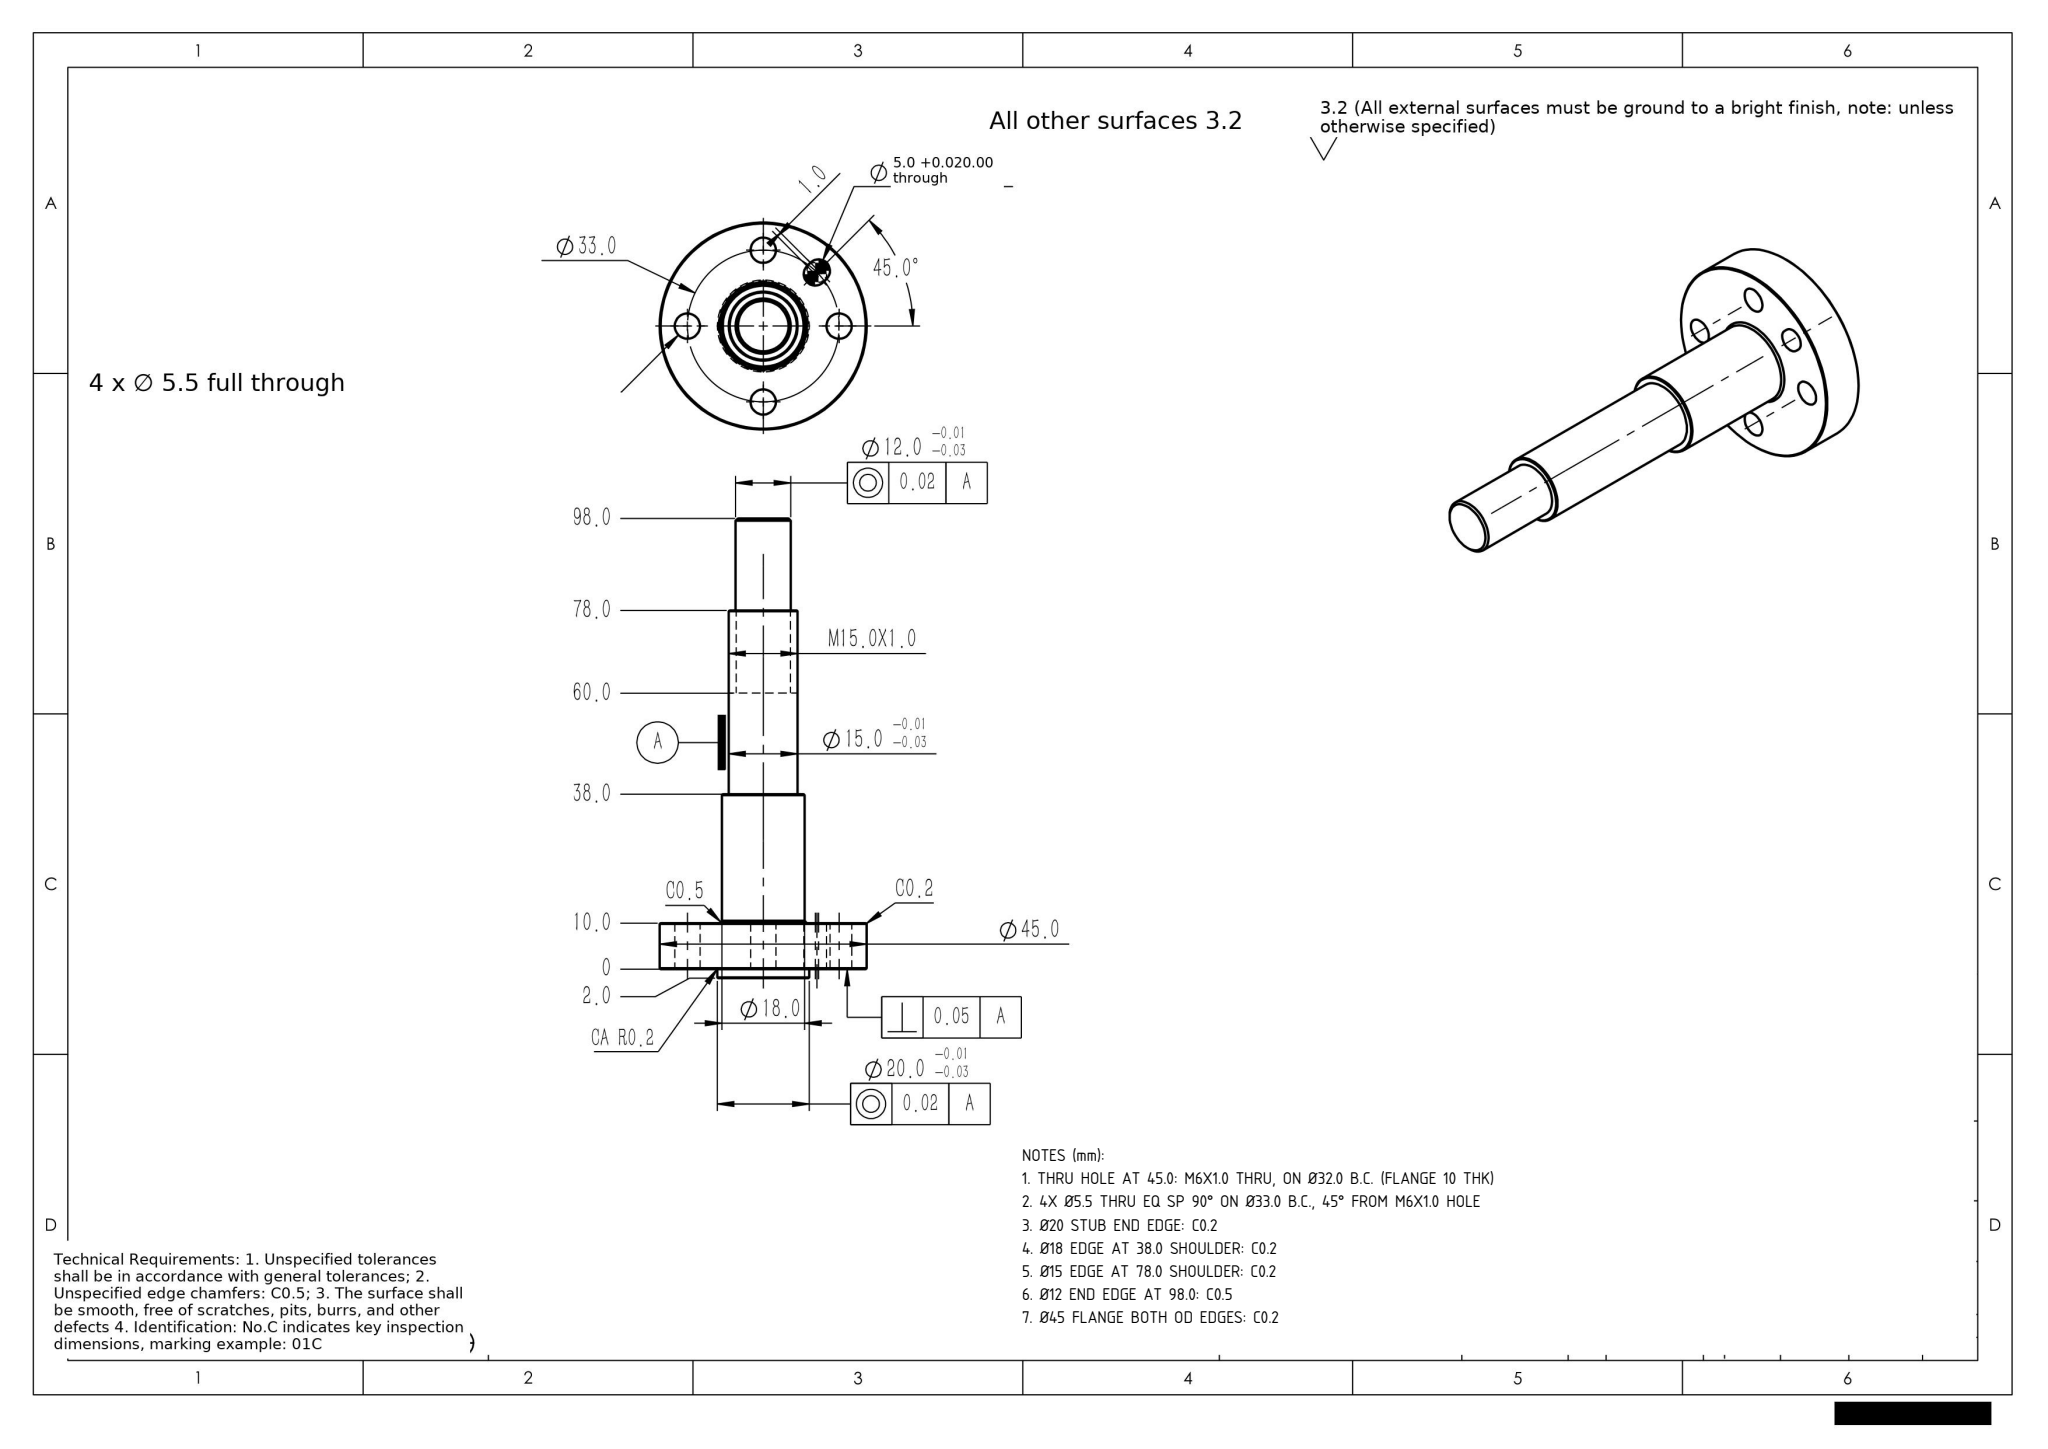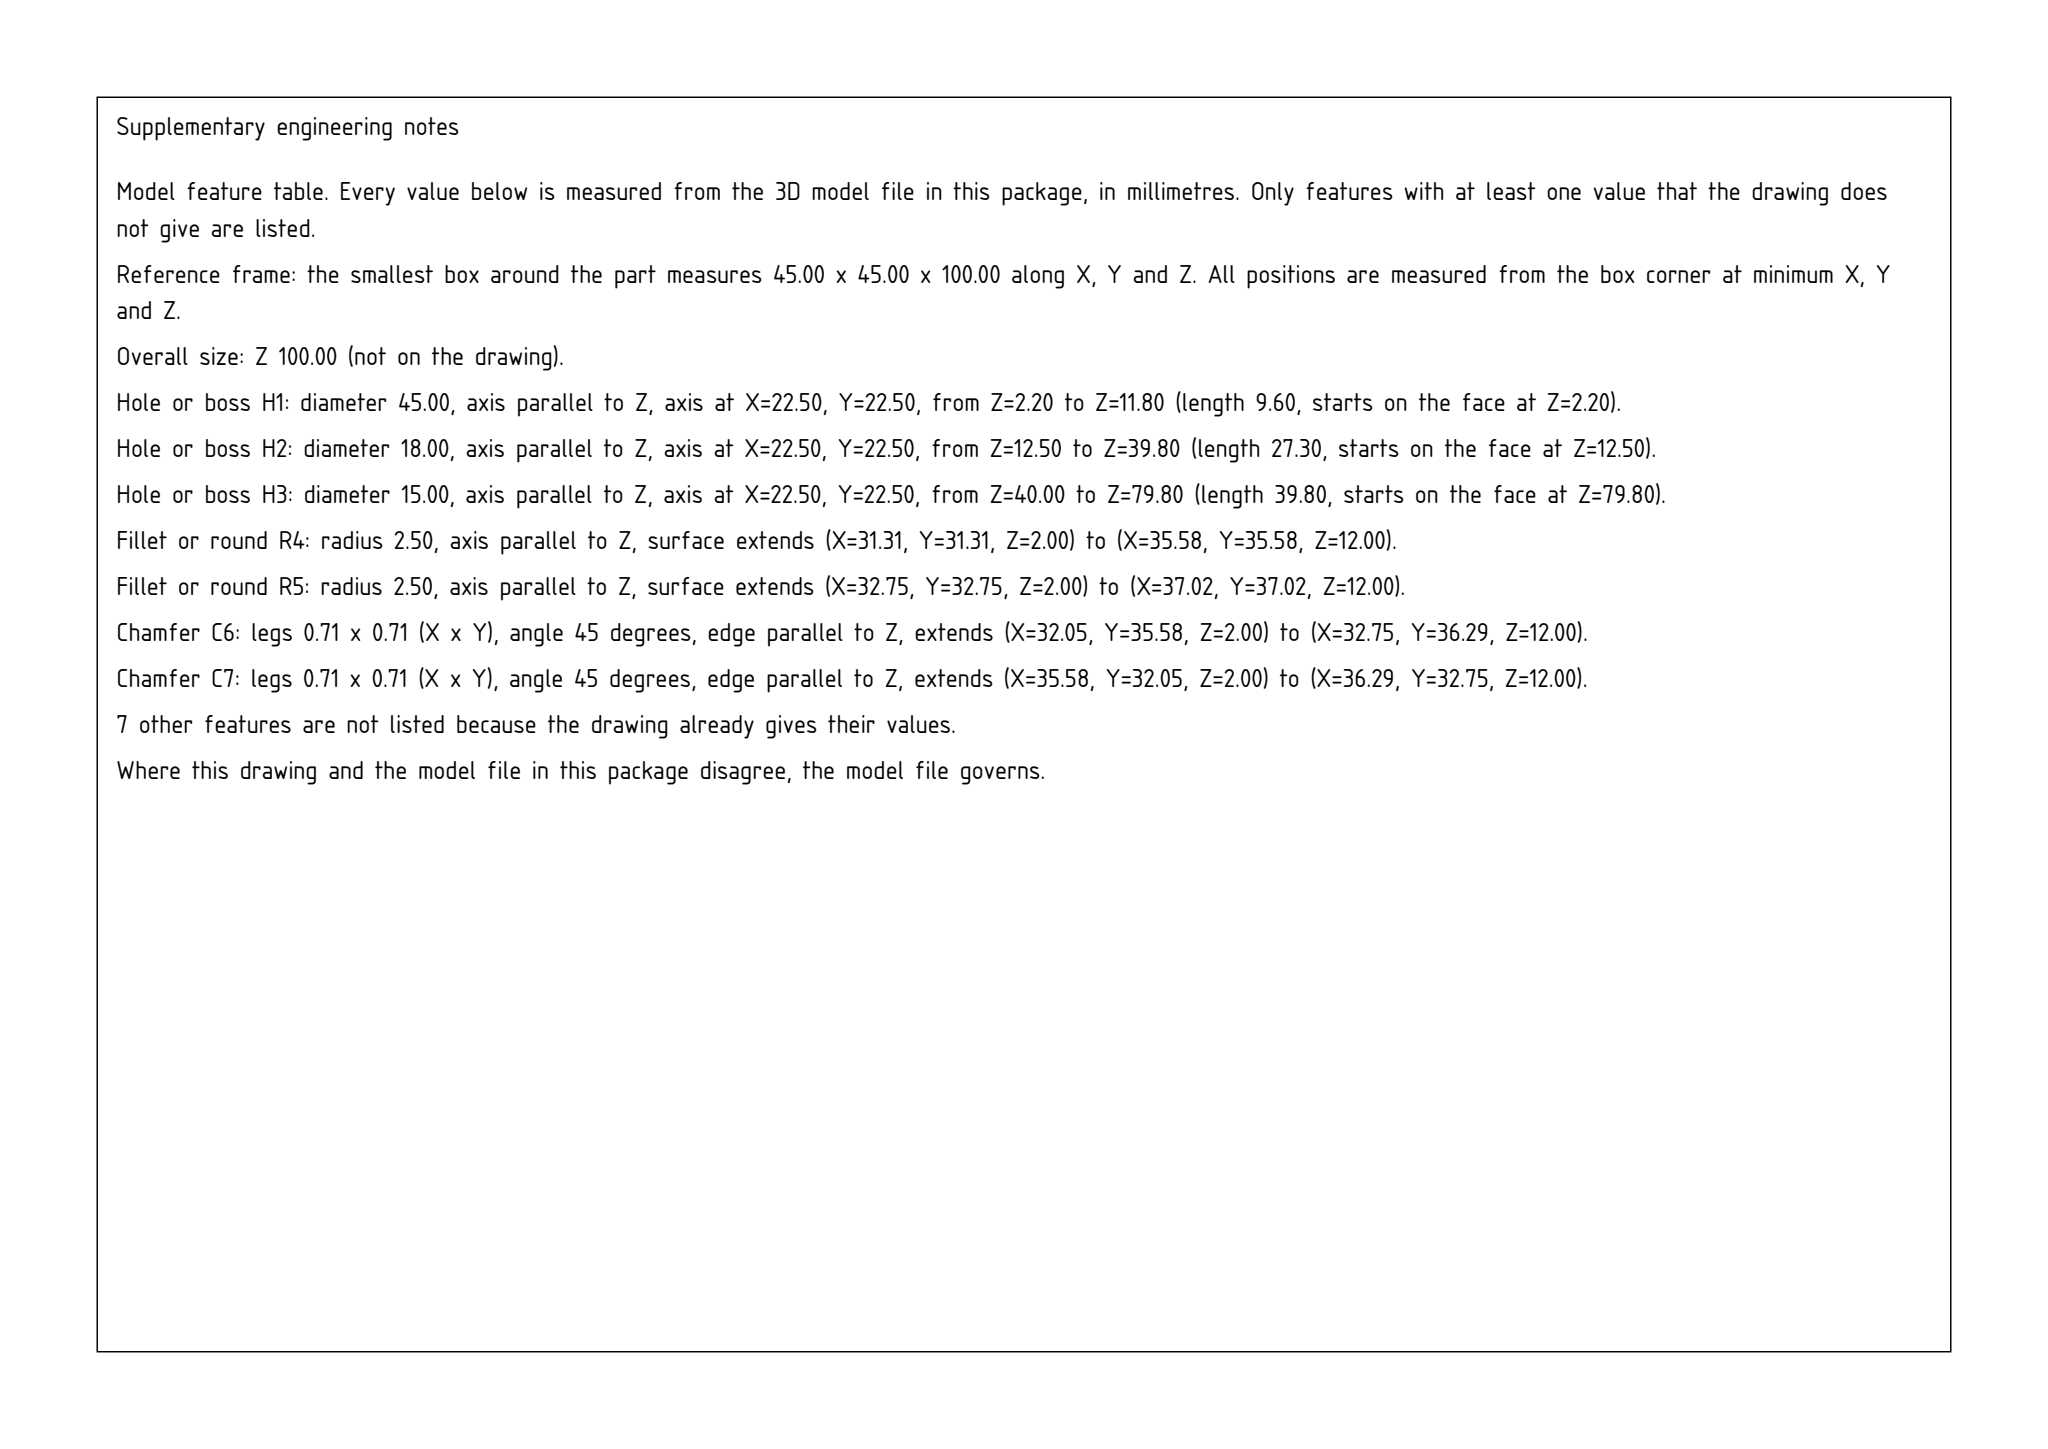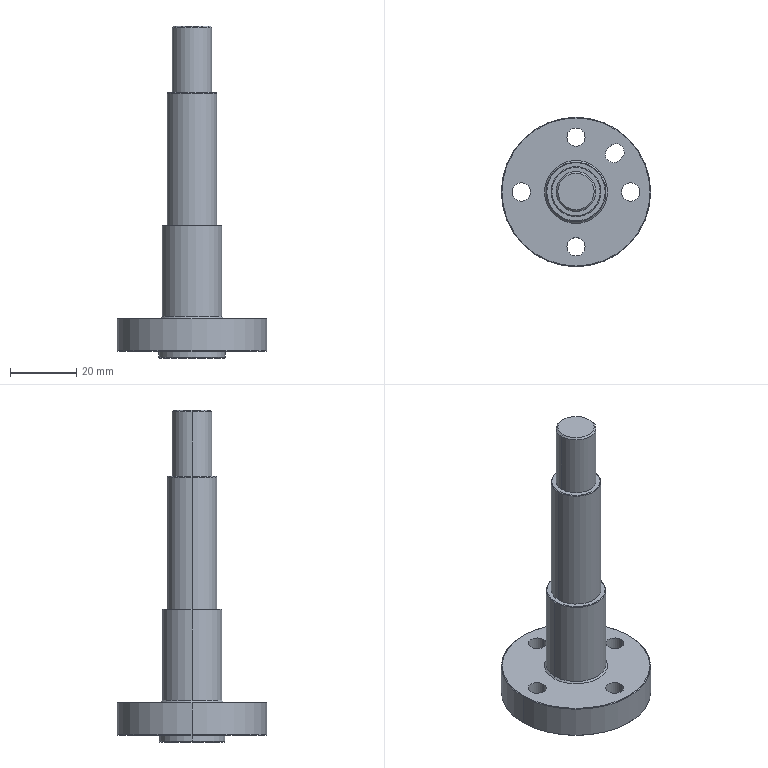Part | SolidWorks | mm | 1 solid | 43 faces | box 45 x 45 x 100 mm | volume 31785 mm3 | cylinder 21 | cone 14 | plane 8 | commonest cylinder face diameters 5.5 x8 5 x3 12 x2 20 x2 15 x2 18 x2 45 x2
Drawing notes:
THRU HOLE AT 45.0: M6X1.0 THRU, ON Ø32.0 B.C. (FLANGE 10 THK) | from the solid: Ø5.0 z-cyl, L=10.0 at (33.81,33.81) = R16.0 @45° from axis (22.5,22.5); paired 5.0 cyl at R17.0 indicates thread feature; leader value 1.0 = pitch
4X Ø5.5 THRU EQ SP 90° ON Ø33.0 B.C., 45° FROM M6X1.0 HOLE | from the solid: Ø5.5 z-cyls L=10.0 at (6.0,22.5),(22.5,6.0),(22.5,39.0),(39.0,22.5): R16.5 (Ø33.0 B.C.) at 0/90/180/270°; M6 hole at 45°
Ø20 STUB END EDGE: C0.2 | from the solid: 90° cone ref dia 19.6 on Ø20 cyl (20-2x0.2); stub L=1.8 of 2.0
Ø18 EDGE AT 38.0 SHOULDER: C0.2 | from the solid: 90° cone ref dia 17.6 at z=40 (Ø18 cyl L=27.3 between 12.5 and 39.8)
Ø15 EDGE AT 78.0 SHOULDER: C0.2 | from the solid: 90° cone ref dia 14.6 at z=80 (Ø15 cyl L=39.8 from z=40)
Ø12 END EDGE AT 98.0: C0.5 | from the solid: 90° cone ref dia 11.0 = 12-2x0.5; Ø12 cyl L=19.5 from z=80 to 99.5
Ø45 FLANGE BOTH OD EDGES: C0.2 | from the solid: 90° cones ref dia 44.6/45.0; Ø45 cyl L=9.6 within 10.0 thk